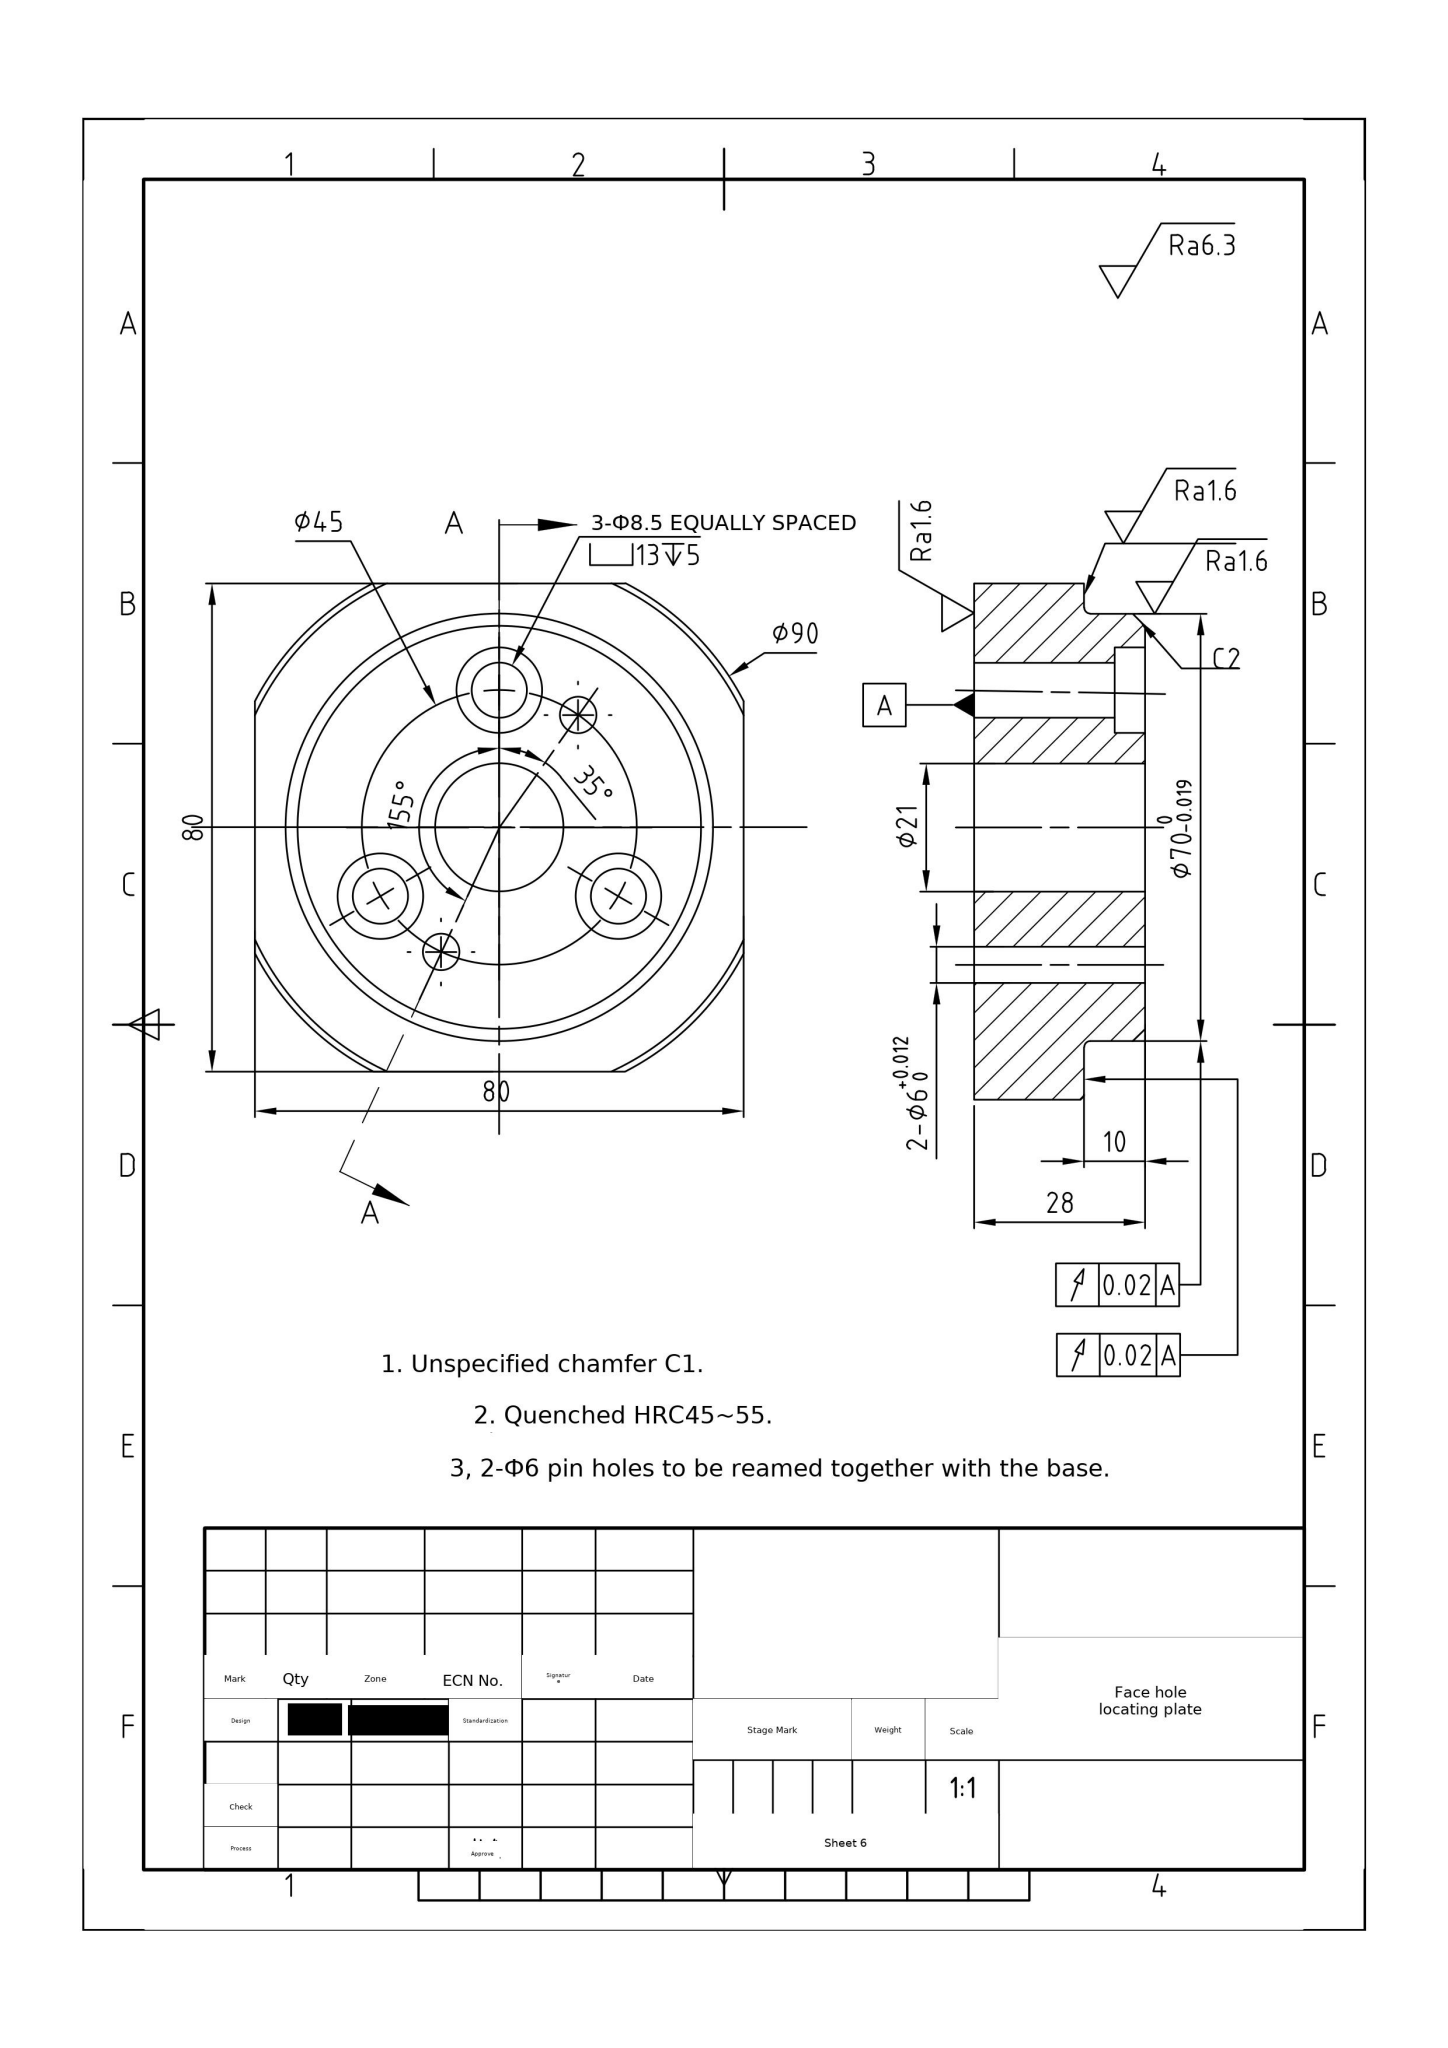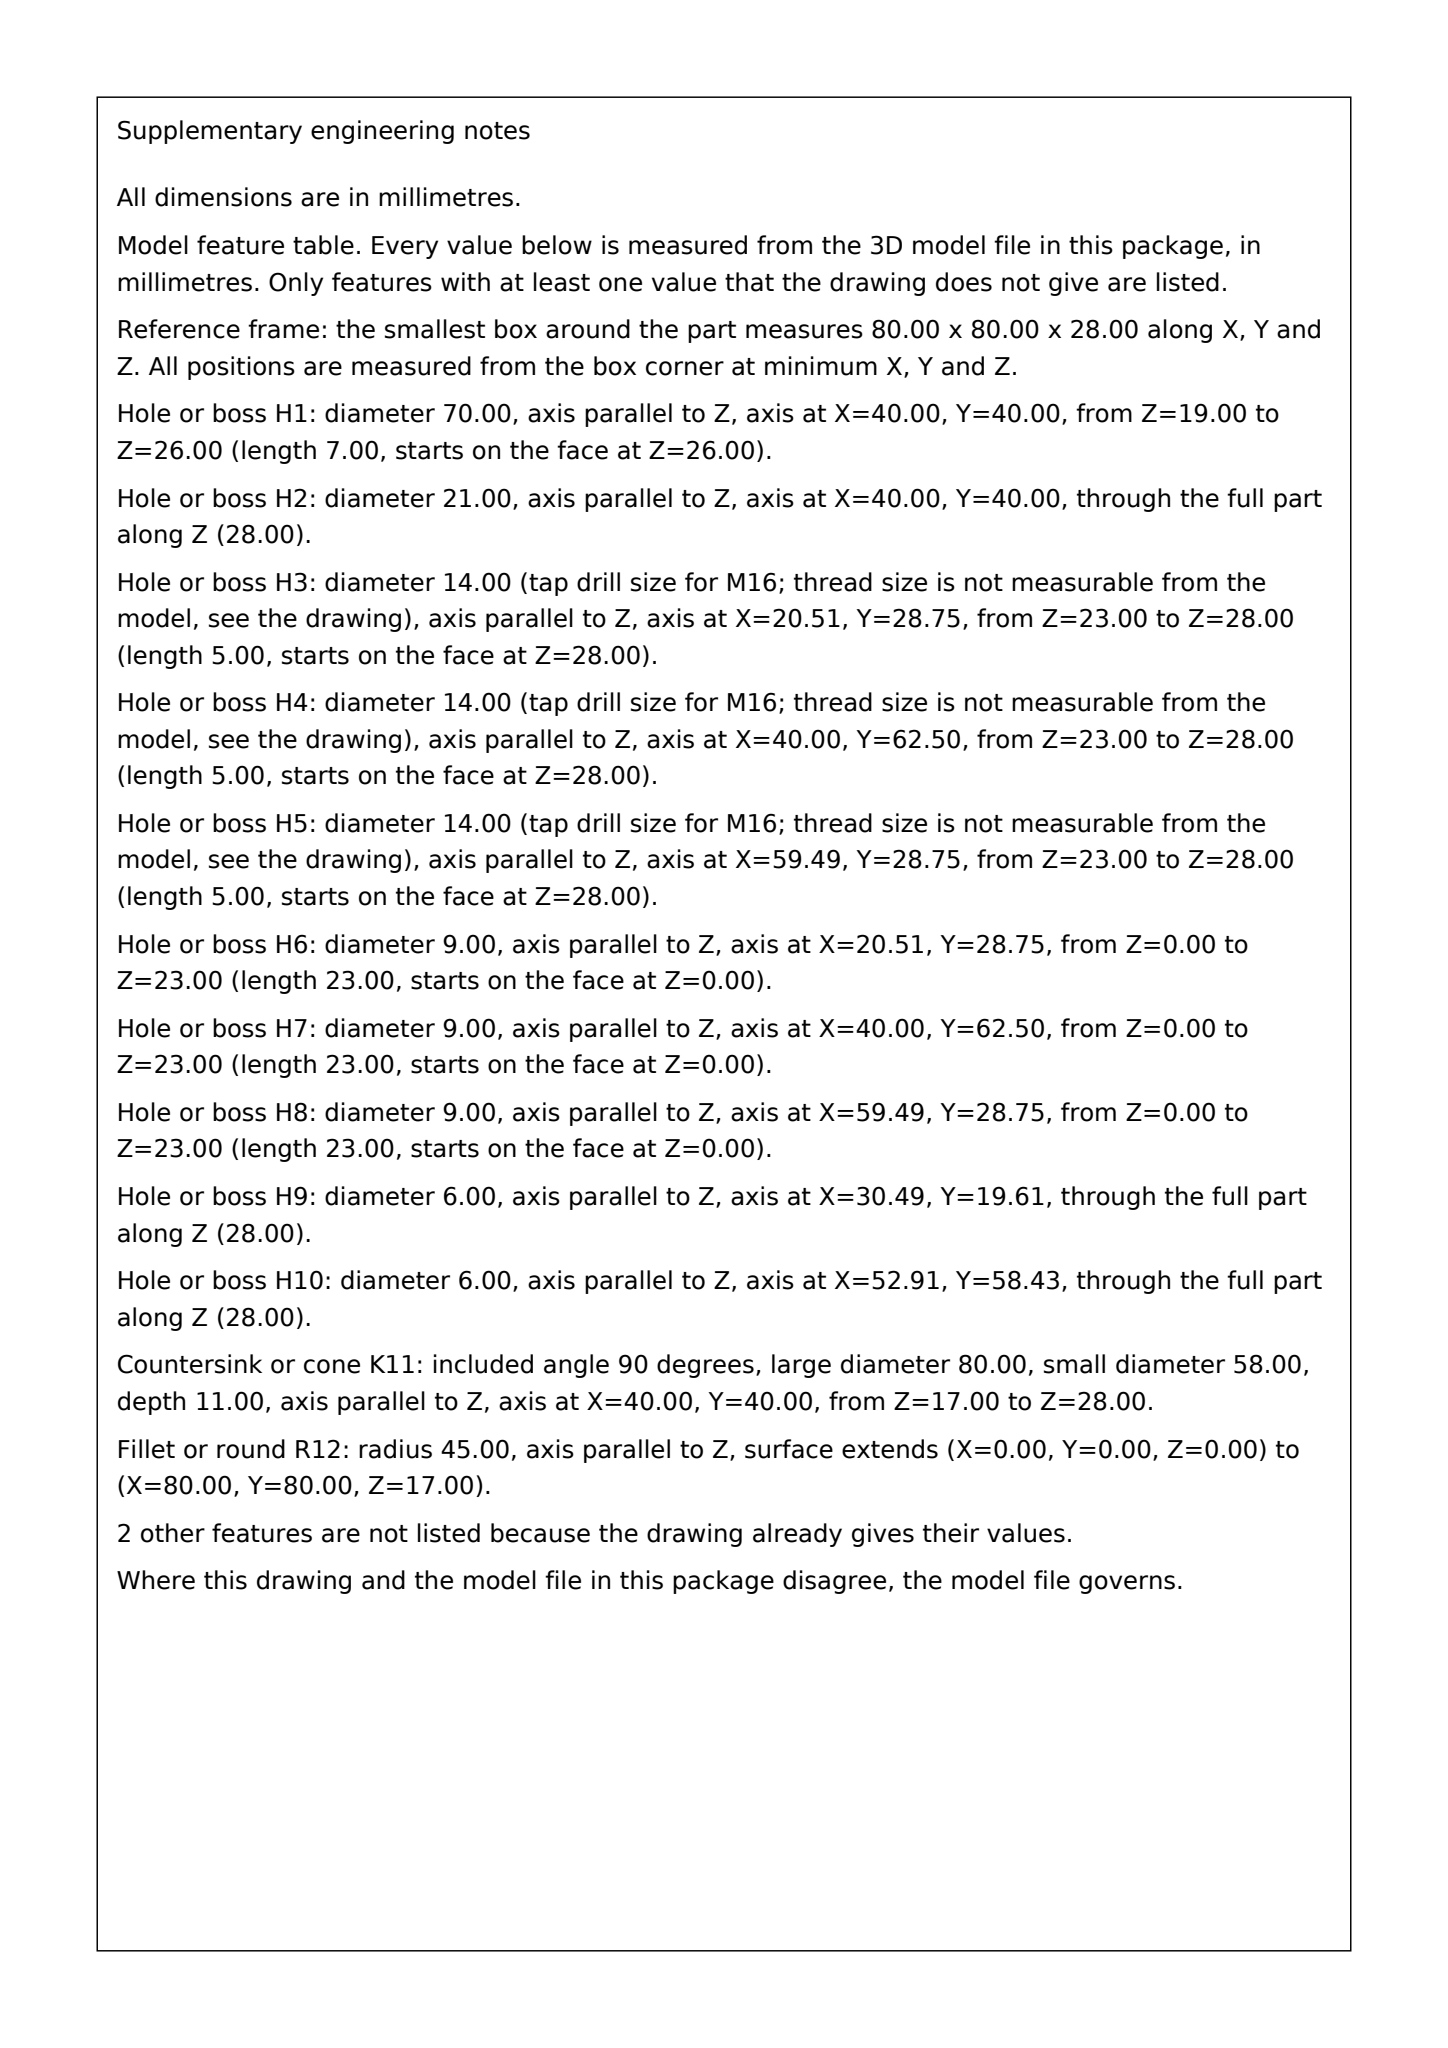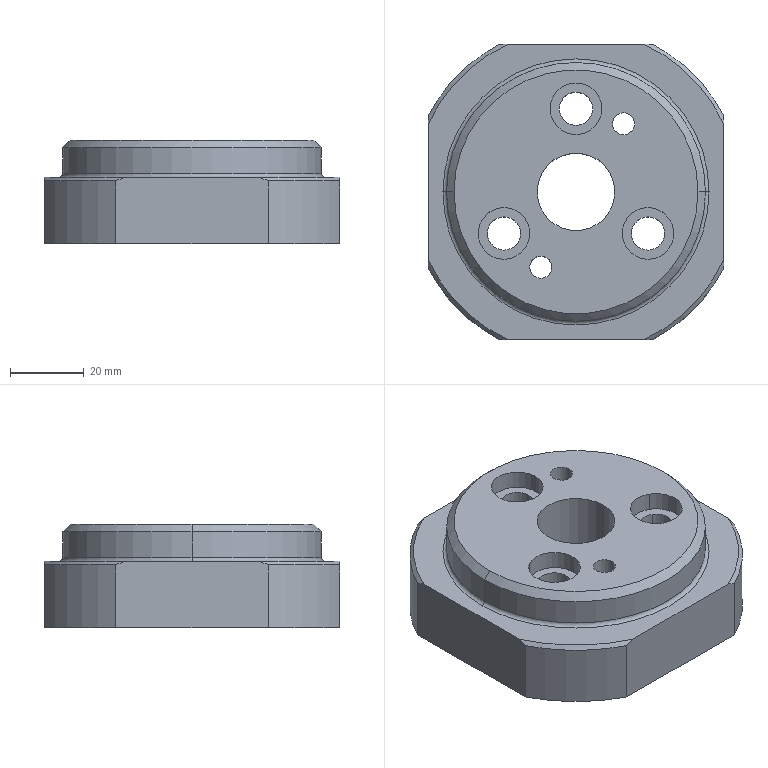Part | SolidWorks | mm | 1 solid | 42 faces | box 80 x 80 x 28 mm | volume 124563 mm3 | cylinder 24 | plane 10 | cone 6 | torus 2 | commonest cylinder face diameters 9 x6 14 x6 6 x4 90 x4 21 x2 70 x2
build123d program:
from build123d import *

# Parameters (mm, degrees)
SKETCH1_R           = 35
BOSS_EXTRUDE1_DEPTH = 10
CHAMFER1_SIZE       = 2
SKETCH2_R           = 45
BOSS_EXTRUDE2_DEPTH = 18
FILLET1_R           = 1
CHAMFER2_SIZE       = 1
SKETCH3_W           = 131.922
SKETCH3_H           = 118.662
SKETCH3_W_2         = 80
SKETCH3_H_2         = 80
CUT_EXTRUDE2_DEPTH  = 67.136
CUT_EXTRUDE3_REACH  = 65.119
SKETCH4_R           = 10.5
SKETCH7_R           = 7
CUT_EXTRUDE4_DEPTH  = 5
CUT_EXTRUDE5_REACH  = 63.066
SKETCH8_R           = 4.5
CIRPATTERN1_COUNT   = 3
CUT_EXTRUDE6_REACH  = 65.119
SKETCH9_R           = 3


with BuildPart() as part:
    # Sketch1 → Boss-Extrude1 (new body)
    with BuildSketch(Plane.XY):
        Circle(SKETCH1_R)
    extrude(amount=BOSS_EXTRUDE1_DEPTH)

    # Chamfer1
    chamfer1_edges = [part.edges().sort_by_distance(p)[0] for p in [
        (-35, 0, 10),
    ]]
    chamfer(chamfer1_edges, length=CHAMFER1_SIZE)

    # Sketch2 → Boss-Extrude2 (add)
    with BuildSketch(Plane(origin=(0, 0, 0), x_dir=(-1, 0, 0), z_dir=(0, 0, -1))):
        Circle(SKETCH2_R)
    extrude(amount=BOSS_EXTRUDE2_DEPTH)

    # Fillet1
    fillet1_edges = [part.edges().sort_by_distance(p)[0] for p in [
        (-35, 0, 0),
    ]]
    fillet(fillet1_edges, radius=FILLET1_R)

    # Chamfer2
    chamfer2_edges = [part.edges().sort_by_distance(p)[0] for p in [
        (45, 0, 0),
    ]]
    chamfer(chamfer2_edges, length=CHAMFER2_SIZE)

    # Sketch3 → Cut-Extrude2 (cut, through all)
    with BuildSketch(Plane.XY):
        Rectangle(SKETCH3_W, SKETCH3_H)
        Rectangle(SKETCH3_W_2, SKETCH3_H_2, mode=Mode.SUBTRACT)
    extrude(amount=-CUT_EXTRUDE2_DEPTH, mode=Mode.SUBTRACT)

    # Sketch4 → Cut-Extrude3 (cut, up to next)
    with BuildSketch(Plane.XY.offset(10), mode=Mode.PRIVATE) as cut_extrude3_sk1:
        Circle(SKETCH4_R)
    cut_extrude3_tool1 = extrude(cut_extrude3_sk1.sketch, amount=-CUT_EXTRUDE3_REACH, mode=Mode.PRIVATE) & part.part
    add(cut_extrude3_tool1.solids().sort_by_distance((0, 0, 10))[0], mode=Mode.SUBTRACT)

    # Sketch7 → Cut-Extrude4 (cut)
    with BuildSketch(Plane.XY.offset(10)):
        with Locations((0, 22.5)):
            Circle(SKETCH7_R)
    cut_extrude4 = extrude(amount=-CUT_EXTRUDE4_DEPTH, mode=Mode.SUBTRACT)

    # Sketch8 → Cut-Extrude5 (cut, up to next)
    with BuildSketch(Plane.XY.offset(5), mode=Mode.PRIVATE) as cut_extrude5_sk1:
        with Locations((0, 22.5)):
            Circle(SKETCH8_R)
    cut_extrude5_tool1 = extrude(cut_extrude5_sk1.sketch, amount=-CUT_EXTRUDE5_REACH, mode=Mode.PRIVATE) & part.part
    cut_extrude5 = cut_extrude5_tool1.solids().sort_by_distance((0, 22.5, 5))[0]
    add(cut_extrude5, mode=Mode.SUBTRACT)

    # CirPattern1: Cut-Extrude4, Cut-Extrude5 ×3 about axis
    cirpattern1_axis = Axis((0, 0, 0), (0, 0, 1))
    add([cut_extrude4.rotate(cirpattern1_axis, i * 360 / CIRPATTERN1_COUNT) for i in range(1, CIRPATTERN1_COUNT)], mode=Mode.SUBTRACT)
    add([cut_extrude5.rotate(cirpattern1_axis, i * 360 / CIRPATTERN1_COUNT) for i in range(1, CIRPATTERN1_COUNT)], mode=Mode.SUBTRACT)

    # Sketch9 → Cut-Extrude6 (cut, up to next)
    with BuildSketch(Plane.XY.offset(10), mode=Mode.PRIVATE) as cut_extrude6_sk1:
        with Locations((-9.509, -20.392)):
            Circle(SKETCH9_R)
    cut_extrude6_tool1 = extrude(cut_extrude6_sk1.sketch, amount=-CUT_EXTRUDE6_REACH, mode=Mode.PRIVATE) & part.part
    # Sketch9 → Cut-Extrude6 (cut, up to next)
    with BuildSketch(Plane.XY.offset(10), mode=Mode.PRIVATE) as cut_extrude6_sk2:
        with Locations((12.905, 18.431)):
            Circle(SKETCH9_R)
    cut_extrude6_tool2 = extrude(cut_extrude6_sk2.sketch, amount=-CUT_EXTRUDE6_REACH, mode=Mode.PRIVATE) & part.part
    add(cut_extrude6_tool1.solids().sort_by_distance((-9.509, -20.392, 10))[0], mode=Mode.SUBTRACT)
    add(cut_extrude6_tool2.solids().sort_by_distance((12.905, 18.431, 10))[0], mode=Mode.SUBTRACT)


solid = part.part